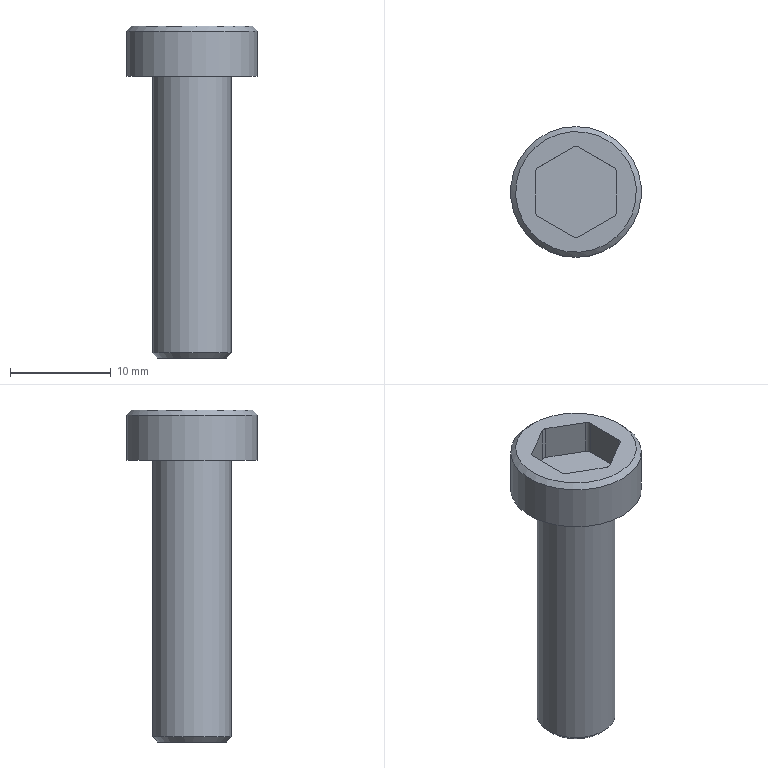Component | NX | SCREW_M8X30 | 1 solid | 20 faces | volume 1795 mm3 | plane 10 | cylinder 8 | cone 2 | commonest cylinder face diameters 1 x6 7.785 x1 13 x1